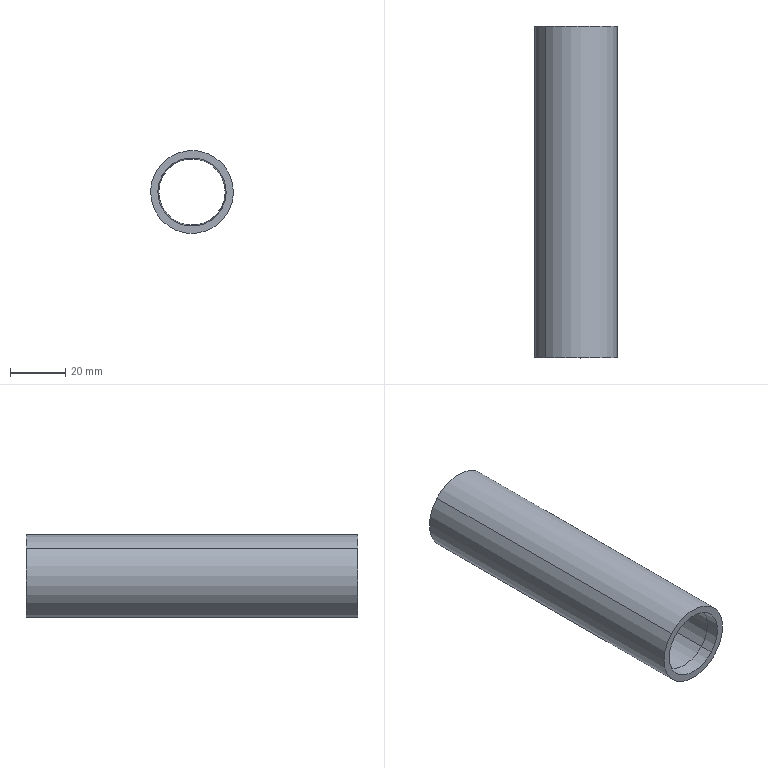Component | SolidWorks | HZ022-A001-D003-1 | 1 solid | 8 faces | box 30 x 120 x 30 mm | volume 30470 mm3 | cylinder 4 | cone 2 | plane 2 | commonest cylinder face diameters 30 x2 24 x2 | material S45C
build123d program:
from build123d import *

# Parameters (mm, degrees)
SKETCH1_2_R           = 15
BOSS_EXTRUDE1_DEPTH   = 120
SKETCH2_R             = 12
CUT_EXTRUDE1_DEPTH    = 122.861
SKETCH1_R             = 12.36
COLLETSEATTAPER_DEPTH = 4.8
COLLETSEATTAPER_DRAFT = -4.289


with BuildPart() as part:
    # Sketch1_2 → Boss-Extrude1 (new body)
    with BuildSketch(Plane(origin=(0, 0, 0), x_dir=(1, 0, 0), z_dir=(0, 1, 0))):
        with Locations(Location((0, 0, 0), (0, 0, 270))):
            Circle(SKETCH1_2_R)
    extrude(amount=BOSS_EXTRUDE1_DEPTH)

    # Sketch2 → Cut-Extrude1 (cut, through all)
    with BuildSketch(Plane(origin=(0, 120, 0), x_dir=(1, 0, 0), z_dir=(0, 1, 0))):
        with Locations(Location((0, 0, 0), (0, 0, 270))):
            Circle(SKETCH2_R)
    extrude(amount=-CUT_EXTRUDE1_DEPTH, mode=Mode.SUBTRACT)


with BuildPart() as colletseattaper_tool:
    # Sketch1 → ColletSeatTaper (with draft: the straight prism first)
    with BuildSketch(Plane.XZ):
        Circle(SKETCH1_R)
    extrude(amount=-COLLETSEATTAPER_DEPTH)
    # ColletSeatTaper: the draft: its side faces are tilted about the plane it starts from
    colletseattaper_sides = [colletseattaper_tool.faces().sort_by_distance(p)[0] for p in [
        (-12.36, 2.4, 0),
    ]]
    draft(colletseattaper_sides, Plane.XZ, COLLETSEATTAPER_DRAFT)


with BuildPart() as part_1:
    add(part.part)

    # ColletSeatTaper: cut by colletseattaper_tool
    add(colletseattaper_tool.part, mode=Mode.SUBTRACT)


solid = part_1.part

# Placed as in the assembly
solid = solid.moved(Location((-12.865, -217.602, 480), (0, 0, 0)))
STEP:
#1=CARTESIAN_POINT('',(-0.156,-8.378,18.581));
#2=VERTEX_POINT('',#1);
#3=CARTESIAN_POINT('',(-0.8569,-8.378,19.214));
#4=VERTEX_POINT('',#3);
#5=CARTESIAN_POINT('',(-0.5065,-8.378,18.898));
#6=DIRECTION('',(0.,-1.,0.));
#7=DIRECTION('',(-0.7418,0.,0.6706));
#8=AXIS2_PLACEMENT_3D('',#5,#6,#7);
#9=CIRCLE('',#8,0.4724);
#10=EDGE_CURVE('',#2,#4,#9,.T.);
#11=ORIENTED_EDGE('',*,*,#10,.F.);
#12=CARTESIAN_POINT('',(-0.1455,-8.567,18.571));
#13=VERTEX_POINT('',#12);
#14=CARTESIAN_POINT('',(-0.1455,-8.567,18.571));
#15=DIRECTION('',(0.05548,-0.9972,-0.05016));
#16=VECTOR('',#15,39.37);
#17=LINE('',#14,#16);
#18=EDGE_CURVE('',#2,#13,#17,.T.);
#19=ORIENTED_EDGE('',*,*,#18,.T.);
#20=CARTESIAN_POINT('',(-0.8675,-8.567,19.224));
#21=VERTEX_POINT('',#20);
#22=CARTESIAN_POINT('',(-0.5065,-8.567,18.898));
#23=DIRECTION('',(0.,-1.,0.));
#24=DIRECTION('',(-0.7418,0.,0.6706));
#25=AXIS2_PLACEMENT_3D('',#22,#23,#24);
#26=CIRCLE('',#25,0.4866);
#27=EDGE_CURVE('',#13,#21,#26,.T.);
#28=ORIENTED_EDGE('',*,*,#27,.T.);
#29=CARTESIAN_POINT('',(-0.8675,-8.567,19.224));
#30=DIRECTION('',(-0.05548,-0.9972,0.05016));
#31=VECTOR('',#30,39.37);
#32=LINE('',#29,#31);
#33=EDGE_CURVE('',#4,#21,#32,.T.);
#34=ORIENTED_EDGE('',*,*,#33,.F.);
#35=EDGE_LOOP('',(#11,#19,#28,#34));
#36=FACE_OUTER_BOUND('',#35,.T.);
#37=CARTESIAN_POINT('',(-0.5065,-8.567,18.898));
#38=DIRECTION('',(0.,-1.,0.));
#39=DIRECTION('',(-0.7418,0.,0.6706));
#40=AXIS2_PLACEMENT_3D('',#37,#38,#39);
#41=CONICAL_SURFACE('',#40,0.4866,0.07486);
#42=ADVANCED_FACE('',(#36),#41,.F.);
#43=CARTESIAN_POINT('',(-0.06843,-3.843,18.502));
#44=VERTEX_POINT('',#43);
#45=CARTESIAN_POINT('',(-0.9446,-3.843,19.294));
#46=VERTEX_POINT('',#45);
#47=CARTESIAN_POINT('',(-0.5065,-3.843,18.898));
#48=DIRECTION('',(0.,1.,0.));
#49=DIRECTION('',(0.7418,0.,-0.6706));
#50=AXIS2_PLACEMENT_3D('',#47,#48,#49);
#51=CIRCLE('',#50,0.5906);
#52=EDGE_CURVE('',#44,#46,#51,.T.);
#53=ORIENTED_EDGE('',*,*,#52,.F.);
#54=CARTESIAN_POINT('',(-0.06843,-8.567,18.502));
#55=VERTEX_POINT('',#54);
#56=CARTESIAN_POINT('',(-0.06843,-3.843,18.502));
#57=DIRECTION('',(0.,-1.,0.));
#58=VECTOR('',#57,39.37);
#59=LINE('',#56,#58);
#60=EDGE_CURVE('',#44,#55,#59,.T.);
#61=ORIENTED_EDGE('',*,*,#60,.T.);
#62=CARTESIAN_POINT('',(-0.9446,-8.567,19.294));
#63=VERTEX_POINT('',#62);
#64=CARTESIAN_POINT('',(-0.5065,-8.567,18.898));
#65=DIRECTION('',(0.,1.,0.));
#66=DIRECTION('',(0.7418,0.,-0.6706));
#67=AXIS2_PLACEMENT_3D('',#64,#65,#66);
#68=CIRCLE('',#67,0.5906);
#69=EDGE_CURVE('',#55,#63,#68,.T.);
#70=ORIENTED_EDGE('',*,*,#69,.T.);
#71=CARTESIAN_POINT('',(-0.9446,-3.843,19.294));
#72=DIRECTION('',(0.,-1.,0.));
#73=VECTOR('',#72,39.37);
#74=LINE('',#71,#73);
#75=EDGE_CURVE('',#46,#63,#74,.T.);
#76=ORIENTED_EDGE('',*,*,#75,.F.);
#77=EDGE_LOOP('',(#53,#61,#70,#76));
#78=FACE_OUTER_BOUND('',#77,.T.);
#79=CARTESIAN_POINT('',(-0.5065,-3.843,18.898));
#80=DIRECTION('',(0.,-1.,0.));
#81=DIRECTION('',(-0.7418,0.,0.6706));
#82=AXIS2_PLACEMENT_3D('',#79,#80,#81);
#83=CYLINDRICAL_SURFACE('',#82,0.5906);
#84=ADVANCED_FACE('',(#78),#83,.T.);
#85=ORIENTED_EDGE('',*,*,#10,.T.);
#86=CARTESIAN_POINT('',(-0.8569,-3.843,19.214));
#87=VERTEX_POINT('',#86);
#88=CARTESIAN_POINT('',(-0.8569,-8.567,19.214));
#89=DIRECTION('',(0.,1.,0.));
#90=VECTOR('',#89,39.37);
#91=LINE('',#88,#90);
#92=EDGE_CURVE('',#4,#87,#91,.T.);
#93=ORIENTED_EDGE('',*,*,#92,.T.);
#94=CARTESIAN_POINT('',(-0.156,-3.843,18.581));
#95=VERTEX_POINT('',#94);
#96=CARTESIAN_POINT('',(-0.5065,-3.843,18.898));
#97=DIRECTION('',(0.,1.,0.));
#98=DIRECTION('',(0.7418,0.,-0.6706));
#99=AXIS2_PLACEMENT_3D('',#96,#97,#98);
#100=CIRCLE('',#99,0.4724);
#101=EDGE_CURVE('',#87,#95,#100,.T.);
#102=ORIENTED_EDGE('',*,*,#101,.T.);
#103=CARTESIAN_POINT('',(-0.156,-8.567,18.581));
#104=DIRECTION('',(0.,1.,0.));
#105=VECTOR('',#104,39.37);
#106=LINE('',#103,#105);
#107=EDGE_CURVE('',#2,#95,#106,.T.);
#108=ORIENTED_EDGE('',*,*,#107,.F.);
#109=EDGE_LOOP('',(#85,#93,#102,#108));
#110=FACE_OUTER_BOUND('',#109,.T.);
#111=CARTESIAN_POINT('',(-0.5065,-8.567,18.898));
#112=DIRECTION('',(0.,1.,0.));
#113=DIRECTION('',(0.7418,0.,-0.6706));
#114=AXIS2_PLACEMENT_3D('',#111,#112,#113);
#115=CYLINDRICAL_SURFACE('',#114,0.4724);
#116=ADVANCED_FACE('',(#110),#115,.F.);
#117=ORIENTED_EDGE('',*,*,#92,.F.);
#118=CARTESIAN_POINT('',(-0.5065,-8.378,18.898));
#119=DIRECTION('',(0.,-1.,0.));
#120=DIRECTION('',(-0.7418,0.,0.6706));
#121=AXIS2_PLACEMENT_3D('',#118,#119,#120);
#122=CIRCLE('',#121,0.4724);
#123=EDGE_CURVE('',#4,#2,#122,.T.);
#124=ORIENTED_EDGE('',*,*,#123,.T.);
#125=ORIENTED_EDGE('',*,*,#107,.T.);
#126=CARTESIAN_POINT('',(-0.5065,-3.843,18.898));
#127=DIRECTION('',(0.,1.,0.));
#128=DIRECTION('',(0.7418,0.,-0.6706));
#129=AXIS2_PLACEMENT_3D('',#126,#127,#128);
#130=CIRCLE('',#129,0.4724);
#131=EDGE_CURVE('',#95,#87,#130,.T.);
#132=ORIENTED_EDGE('',*,*,#131,.T.);
#133=EDGE_LOOP('',(#117,#124,#125,#132));
#134=FACE_OUTER_BOUND('',#133,.T.);
#135=CARTESIAN_POINT('',(-0.5065,-8.567,18.898));
#136=DIRECTION('',(0.,1.,0.));
#137=DIRECTION('',(0.7418,0.,-0.6706));
#138=AXIS2_PLACEMENT_3D('',#135,#136,#137);
#139=CYLINDRICAL_SURFACE('',#138,0.4724);
#140=ADVANCED_FACE('',(#134),#139,.F.);
#141=ORIENTED_EDGE('',*,*,#60,.F.);
#142=CARTESIAN_POINT('',(-0.5065,-3.843,18.898));
#143=DIRECTION('',(0.,1.,0.));
#144=DIRECTION('',(0.7418,0.,-0.6706));
#145=AXIS2_PLACEMENT_3D('',#142,#143,#144);
#146=CIRCLE('',#145,0.5906);
#147=EDGE_CURVE('',#46,#44,#146,.T.);
#148=ORIENTED_EDGE('',*,*,#147,.F.);
#149=ORIENTED_EDGE('',*,*,#75,.T.);
#150=CARTESIAN_POINT('',(-0.5065,-8.567,18.898));
#151=DIRECTION('',(0.,1.,0.));
#152=DIRECTION('',(0.7418,0.,-0.6706));
#153=AXIS2_PLACEMENT_3D('',#150,#151,#152);
#154=CIRCLE('',#153,0.5906);
#155=EDGE_CURVE('',#63,#55,#154,.T.);
#156=ORIENTED_EDGE('',*,*,#155,.T.);
#157=EDGE_LOOP('',(#141,#148,#149,#156));
#158=FACE_OUTER_BOUND('',#157,.T.);
#159=CARTESIAN_POINT('',(-0.5065,-3.843,18.898));
#160=DIRECTION('',(0.,-1.,0.));
#161=DIRECTION('',(-0.7418,0.,0.6706));
#162=AXIS2_PLACEMENT_3D('',#159,#160,#161);
#163=CYLINDRICAL_SURFACE('',#162,0.5906);
#164=ADVANCED_FACE('',(#158),#163,.T.);
#165=ORIENTED_EDGE('',*,*,#131,.F.);
#166=ORIENTED_EDGE('',*,*,#101,.F.);
#167=EDGE_LOOP('',(#165,#166));
#168=FACE_BOUND('',#167,.T.);
#169=ORIENTED_EDGE('',*,*,#147,.T.);
#170=ORIENTED_EDGE('',*,*,#52,.T.);
#171=EDGE_LOOP('',(#169,#170));
#172=FACE_OUTER_BOUND('',#171,.T.);
#173=CARTESIAN_POINT('',(-0.5065,-3.843,18.898));
#174=DIRECTION('',(0.,1.,0.));
#175=DIRECTION('',(0.7418,0.,-0.6706));
#176=AXIS2_PLACEMENT_3D('',#173,#174,#175);
#177=PLANE('',#176);
#178=ADVANCED_FACE('',(#168,#172),#177,.T.);
#179=CARTESIAN_POINT('',(-0.5065,-8.567,18.898));
#180=DIRECTION('',(0.,-1.,0.));
#181=DIRECTION('',(-0.7418,0.,0.6706));
#182=AXIS2_PLACEMENT_3D('',#179,#180,#181);
#183=CIRCLE('',#182,0.4866);
#184=EDGE_CURVE('',#21,#13,#183,.T.);
#185=ORIENTED_EDGE('',*,*,#184,.F.);
#186=ORIENTED_EDGE('',*,*,#27,.F.);
#187=EDGE_LOOP('',(#185,#186));
#188=FACE_BOUND('',#187,.T.);
#189=ORIENTED_EDGE('',*,*,#155,.F.);
#190=ORIENTED_EDGE('',*,*,#69,.F.);
#191=EDGE_LOOP('',(#189,#190));
#192=FACE_OUTER_BOUND('',#191,.T.);
#193=CARTESIAN_POINT('',(-0.5065,-8.567,18.898));
#194=DIRECTION('',(0.,1.,0.));
#195=DIRECTION('',(0.7418,0.,-0.6706));
#196=AXIS2_PLACEMENT_3D('',#193,#194,#195);
#197=PLANE('',#196);
#198=ADVANCED_FACE('',(#188,#192),#197,.F.);
#199=ORIENTED_EDGE('',*,*,#18,.F.);
#200=ORIENTED_EDGE('',*,*,#123,.F.);
#201=ORIENTED_EDGE('',*,*,#33,.T.);
#202=ORIENTED_EDGE('',*,*,#184,.T.);
#203=EDGE_LOOP('',(#199,#200,#201,#202));
#204=FACE_OUTER_BOUND('',#203,.T.);
#205=CARTESIAN_POINT('',(-0.5065,-8.567,18.898));
#206=DIRECTION('',(0.,-1.,0.));
#207=DIRECTION('',(-0.7418,0.,0.6706));
#208=AXIS2_PLACEMENT_3D('',#205,#206,#207);
#209=CONICAL_SURFACE('',#208,0.4866,0.07486);
#210=ADVANCED_FACE('',(#204),#209,.F.);
#211=CLOSED_SHELL('',(#42,#84,#116,#140,#164,#178,#198,#210));
#212=MANIFOLD_SOLID_BREP('',#211);
#213=CARTESIAN_POINT('',(0.,0.,0.));
#214=DIRECTION('',(0.,0.,1.));
#215=DIRECTION('',(1.,0.,0.));
#216=AXIS2_PLACEMENT_3D('',#213,#214,#215);
#217=(LENGTH_UNIT()NAMED_UNIT(*)SI_UNIT($,.METRE.));
#218=LENGTH_MEASURE_WITH_UNIT(LENGTH_MEASURE(0.0254),#217);
#219=DIMENSIONAL_EXPONENTS(1.,0.,0.,0.,0.,0.,0.);
#220=(CONVERSION_BASED_UNIT('',#218)LENGTH_UNIT()NAMED_UNIT(#219));
#221=UNCERTAINTY_MEASURE_WITH_UNIT(LENGTH_MEASURE(0.00001),#220,'','');
#222=(NAMED_UNIT(*)PLANE_ANGLE_UNIT()SI_UNIT($,.RADIAN.));
#223=(NAMED_UNIT(*)SI_UNIT($,.STERADIAN.)SOLID_ANGLE_UNIT());
#224=(GEOMETRIC_REPRESENTATION_CONTEXT(3)GLOBAL_UNCERTAINTY_ASSIGNED_CONTEXT((#221))GLOBAL_UNIT_ASSIGNED_CONTEXT((#220,#222,#223))REPRESENTATION_CONTEXT('',''));
#225=ADVANCED_BREP_SHAPE_REPRESENTATION('',(#212,#216),#224);
#226=COLOUR_RGB('',0.7922,0.8196,0.9333);
#227=FILL_AREA_STYLE_COLOUR('',#226);
#228=FILL_AREA_STYLE('',(#227));
#229=SURFACE_STYLE_FILL_AREA(#228);
#230=SURFACE_SIDE_STYLE('',(#229));
#231=SURFACE_STYLE_USAGE(.BOTH.,#230);
#232=PRESENTATION_STYLE_ASSIGNMENT((#231));
#233=STYLED_ITEM('',(#232),#212);
#234=PRESENTATION_LAYER_ASSIGNMENT('','',(#233));
#235=(LENGTH_UNIT()NAMED_UNIT(*)SI_UNIT($,.METRE.));
#236=LENGTH_MEASURE_WITH_UNIT(LENGTH_MEASURE(0.0254),#235);
#237=DIMENSIONAL_EXPONENTS(1.,0.,0.,0.,0.,0.,0.);
#238=(CONVERSION_BASED_UNIT('',#236)LENGTH_UNIT()NAMED_UNIT(#237));
#239=UNCERTAINTY_MEASURE_WITH_UNIT(LENGTH_MEASURE(0.00001),#238,'','');
#240=(NAMED_UNIT(*)PLANE_ANGLE_UNIT()SI_UNIT($,.RADIAN.));
#241=(NAMED_UNIT(*)SI_UNIT($,.STERADIAN.)SOLID_ANGLE_UNIT());
#242=(GEOMETRIC_REPRESENTATION_CONTEXT(3)GLOBAL_UNCERTAINTY_ASSIGNED_CONTEXT((#239))GLOBAL_UNIT_ASSIGNED_CONTEXT((#238,#240,#241))REPRESENTATION_CONTEXT('',''));
#243=MECHANICAL_DESIGN_GEOMETRIC_PRESENTATION_REPRESENTATION('',(#233),#242);